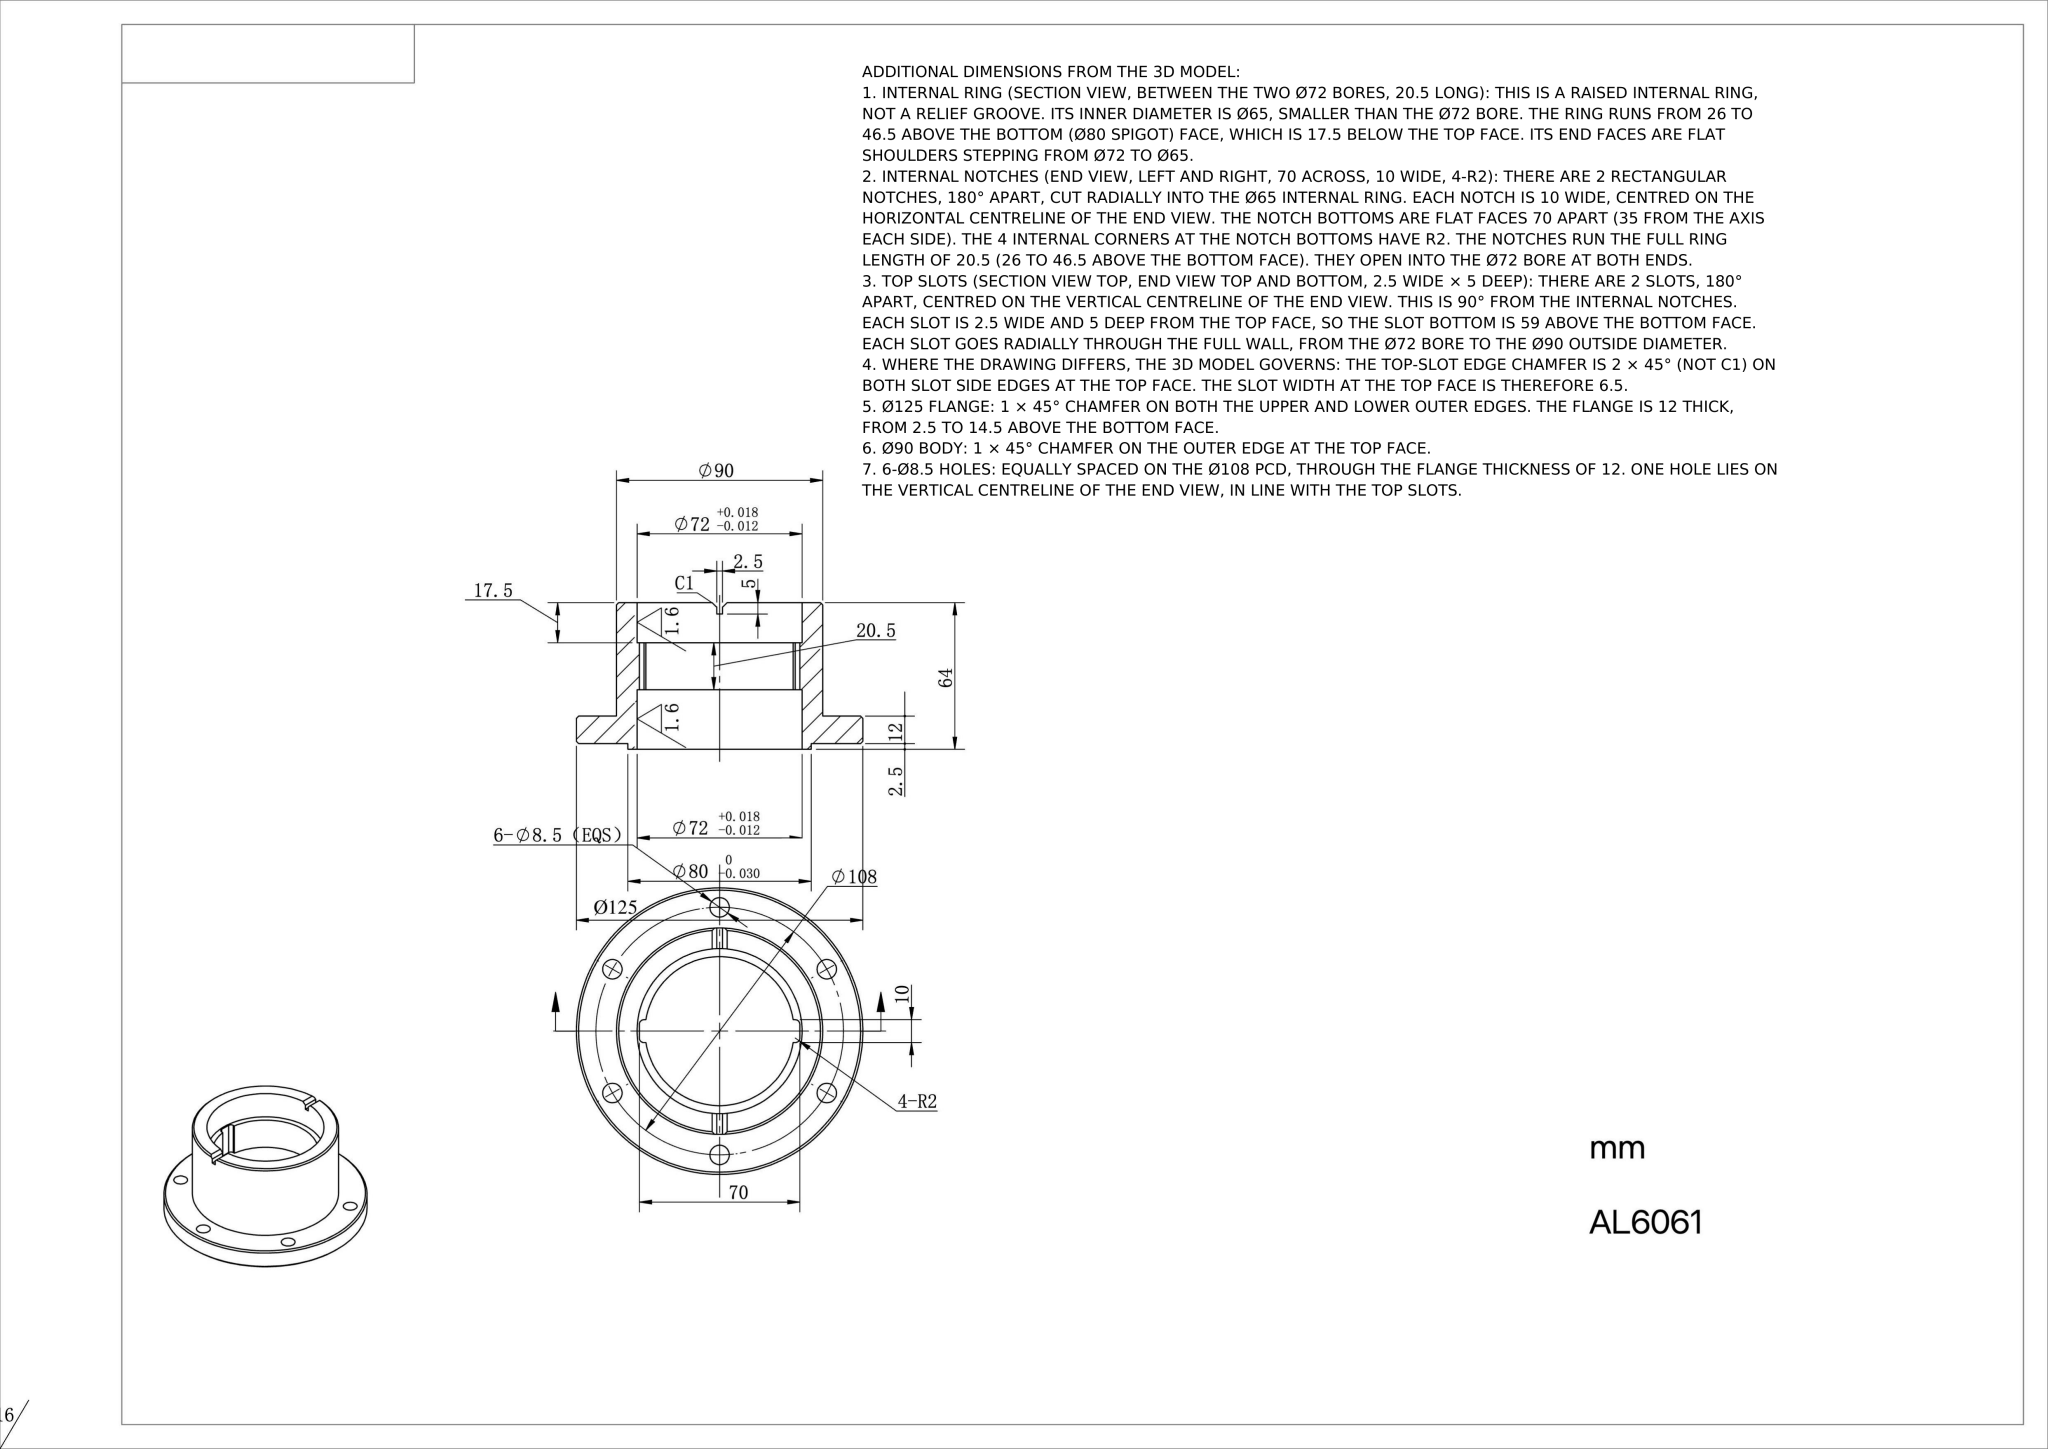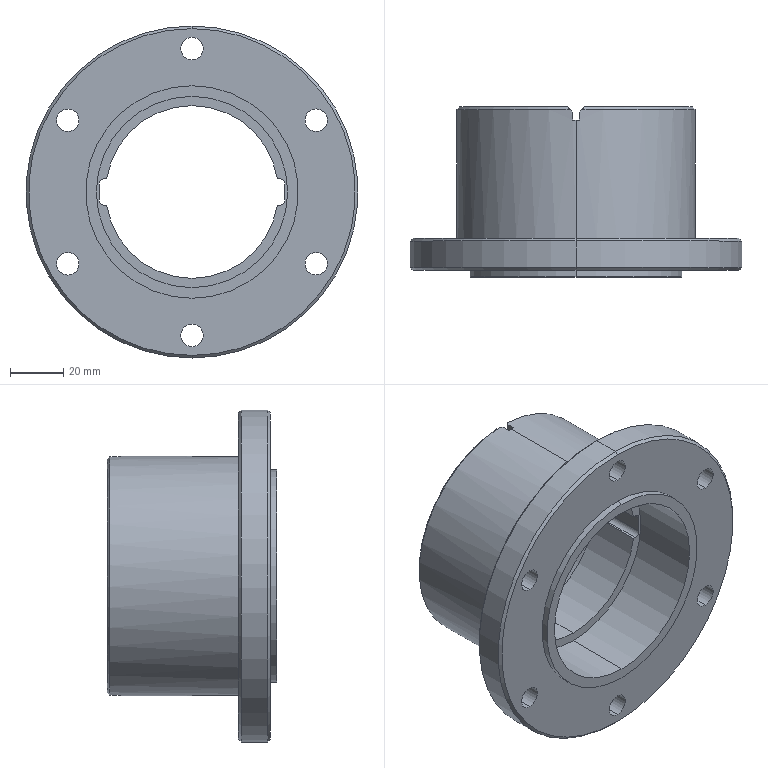Part | NX | mm | Keyed Flanged Bushing | 1 solid | 58 faces | box 125 x 64 x 125 mm | volume 223683 mm3 | cylinder 29 | plane 23 | cone 6 | commonest cylinder face diameters 8.5 x12 72 x4 4 x4 65 x3 125 x2 90 x2 80 x2